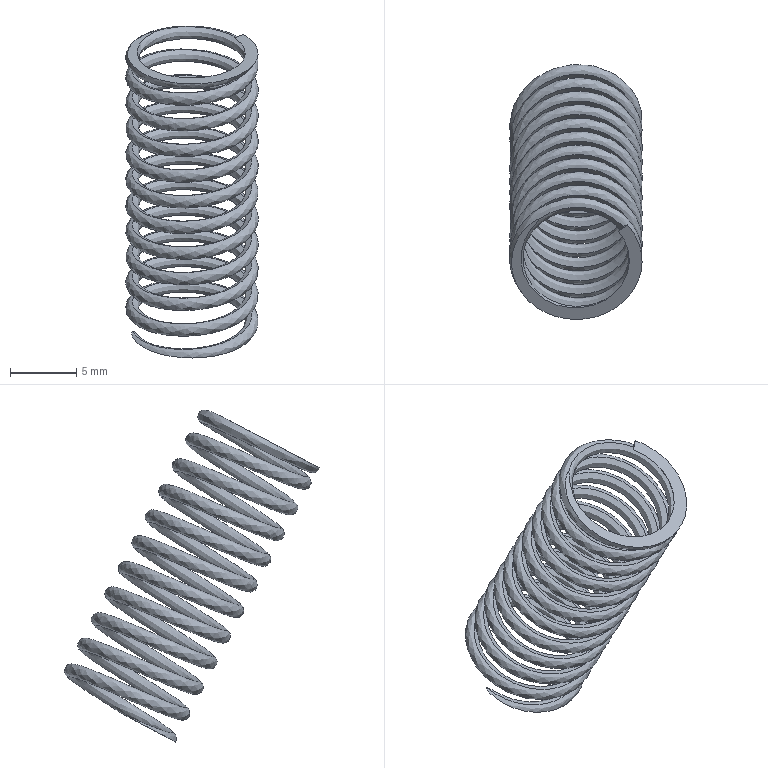Component | SolidWorks | Spring-3 | 1 solid | 5 faces | volume 246 mm3 | plane 3 | spline 2